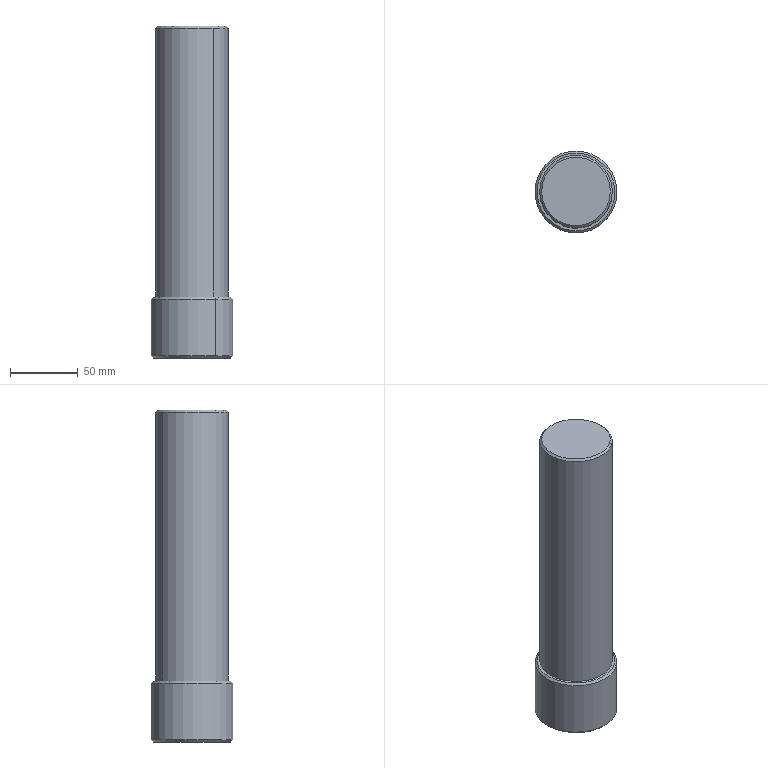Component | SolidWorks | PunchMandrel-1 | 1 solid | 13 faces | box 60.5 x 60.5 x 245 mm | volume 580883 mm3 | cone 6 | cylinder 4 | plane 3 | commonest cylinder face diameters 53.65 x2 60.5 x2
build123d program:
from build123d import *

# Parameters (mm, degrees)
CHAMFER1_SIZE = 1.5


with BuildPart() as part:
    # Sketch1 → Revolve1 (revolve)
    with BuildSketch(Plane.XY, mode=Mode.PRIVATE) as revolve1_sk:
        Polygon((0, 0), (0, 245), (30.25, 245), (30.25, 200), (26.825, 200), (26.825, 0), align=None)
    revolve(revolve1_sk.sketch.rotate(Axis((0, 0, 0), (0, 1, 0)), 90), axis=Axis((0, 0, 0), (0, 1, 0)))

    # Chamfer1
    chamfer1_edges = [part.edges().sort_by_distance(p)[0] for p in [
        (0, 0, 26.825),
        (0, 200, 30.25),
        (0, 245, 30.25),
    ]]
    chamfer(chamfer1_edges, length=CHAMFER1_SIZE)


solid = part.part

# Placed as in the assembly
solid = solid.moved(Location((0, 0, -1), (-90, 0, 0)))
STEP:
#1=COLOUR_RGB('',0.7922,0.8196,0.9333);
#2=FILL_AREA_STYLE_COLOUR('',#1);
#3=FILL_AREA_STYLE('',(#2));
#4=SURFACE_STYLE_FILL_AREA(#3);
#5=SURFACE_SIDE_STYLE('',(#4));
#6=SURFACE_STYLE_USAGE(.BOTH.,#5);
#7=PRESENTATION_STYLE_ASSIGNMENT((#6));
#8=CARTESIAN_POINT('',(0.6561,-0.9223,-7.913));
#9=VERTEX_POINT('',#8);
#10=CARTESIAN_POINT('',(-0.6561,0.9223,-7.913));
#11=VERTEX_POINT('',#10);
#12=CARTESIAN_POINT('',(-0.,-0.,-7.913));
#13=DIRECTION('',(0.,0.,1.));
#14=DIRECTION('',(0.5797,-0.8148,0.));
#15=AXIS2_PLACEMENT_3D('',#12,#13,#14);
#16=CIRCLE('',#15,1.132);
#17=EDGE_CURVE('',#9,#11,#16,.T.);
#18=ORIENTED_EDGE('',*,*,#17,.F.);
#19=CARTESIAN_POINT('',(0.6904,-0.9704,-7.972));
#20=VERTEX_POINT('',#19);
#21=CARTESIAN_POINT('',(0.6561,-0.9223,-7.913));
#22=DIRECTION('',(0.4099,-0.5762,-0.7071));
#23=VECTOR('',#22,39.37);
#24=LINE('',#21,#23);
#25=EDGE_CURVE('',#9,#20,#24,.T.);
#26=ORIENTED_EDGE('',*,*,#25,.T.);
#27=CARTESIAN_POINT('',(-0.6904,0.9704,-7.972));
#28=VERTEX_POINT('',#27);
#29=CARTESIAN_POINT('',(-0.,-0.,-7.972));
#30=DIRECTION('',(-0.,-0.,-1.));
#31=DIRECTION('',(0.5797,-0.8148,0.));
#32=AXIS2_PLACEMENT_3D('',#29,#30,#31);
#33=CIRCLE('',#32,1.191);
#34=EDGE_CURVE('',#28,#20,#33,.T.);
#35=ORIENTED_EDGE('',*,*,#34,.F.);
#36=CARTESIAN_POINT('',(-0.6561,0.9223,-7.913));
#37=DIRECTION('',(-0.4099,0.5762,-0.7071));
#38=VECTOR('',#37,39.37);
#39=LINE('',#36,#38);
#40=EDGE_CURVE('',#11,#28,#39,.T.);
#41=ORIENTED_EDGE('',*,*,#40,.F.);
#42=EDGE_LOOP('',(#18,#26,#35,#41));
#43=FACE_OUTER_BOUND('',#42,.T.);
#44=CARTESIAN_POINT('',(-0.,-0.,-7.913));
#45=DIRECTION('',(-0.,-0.,-1.));
#46=DIRECTION('',(-0.5797,0.8148,0.));
#47=AXIS2_PLACEMENT_3D('',#44,#45,#46);
#48=CONICAL_SURFACE('',#47,1.132,0.7854);
#49=ADVANCED_FACE('',(#43),#48,.T.);
#50=CARTESIAN_POINT('',(-0.6561,0.9223,-9.685));
#51=VERTEX_POINT('',#50);
#52=CARTESIAN_POINT('',(0.6561,-0.9223,-9.685));
#53=VERTEX_POINT('',#52);
#54=CARTESIAN_POINT('',(-0.,-0.,-9.685));
#55=DIRECTION('',(-0.,-0.,-1.));
#56=DIRECTION('',(-0.5797,0.8148,0.));
#57=AXIS2_PLACEMENT_3D('',#54,#55,#56);
#58=CIRCLE('',#57,1.132);
#59=EDGE_CURVE('',#51,#53,#58,.T.);
#60=ORIENTED_EDGE('',*,*,#59,.F.);
#61=CARTESIAN_POINT('',(-0.6904,0.9704,-9.626));
#62=VERTEX_POINT('',#61);
#63=CARTESIAN_POINT('',(-0.6904,0.9704,-9.626));
#64=DIRECTION('',(-0.4099,0.5762,0.7071));
#65=VECTOR('',#64,39.37);
#66=LINE('',#63,#65);
#67=EDGE_CURVE('',#51,#62,#66,.T.);
#68=ORIENTED_EDGE('',*,*,#67,.T.);
#69=CARTESIAN_POINT('',(0.6904,-0.9704,-9.626));
#70=VERTEX_POINT('',#69);
#71=CARTESIAN_POINT('',(-0.,-0.,-9.626));
#72=DIRECTION('',(0.,0.,1.));
#73=DIRECTION('',(-0.5797,0.8148,0.));
#74=AXIS2_PLACEMENT_3D('',#71,#72,#73);
#75=CIRCLE('',#74,1.191);
#76=EDGE_CURVE('',#70,#62,#75,.T.);
#77=ORIENTED_EDGE('',*,*,#76,.F.);
#78=CARTESIAN_POINT('',(0.6904,-0.9704,-9.626));
#79=DIRECTION('',(0.4099,-0.5762,0.7071));
#80=VECTOR('',#79,39.37);
#81=LINE('',#78,#80);
#82=EDGE_CURVE('',#53,#70,#81,.T.);
#83=ORIENTED_EDGE('',*,*,#82,.F.);
#84=EDGE_LOOP('',(#60,#68,#77,#83));
#85=FACE_OUTER_BOUND('',#84,.T.);
#86=CARTESIAN_POINT('',(-0.,-0.,-9.626));
#87=DIRECTION('',(0.,0.,1.));
#88=DIRECTION('',(0.5797,-0.8148,0.));
#89=AXIS2_PLACEMENT_3D('',#86,#87,#88);
#90=CONICAL_SURFACE('',#89,1.191,0.7854);
#91=ADVANCED_FACE('',(#85),#90,.T.);
#92=CARTESIAN_POINT('',(0.578,-0.8124,-0.03937));
#93=VERTEX_POINT('',#92);
#94=CARTESIAN_POINT('',(-0.578,0.8124,-0.03937));
#95=VERTEX_POINT('',#94);
#96=CARTESIAN_POINT('',(-0.,0.,-0.03937));
#97=DIRECTION('',(0.,0.,1.));
#98=DIRECTION('',(0.5797,-0.8148,0.));
#99=AXIS2_PLACEMENT_3D('',#96,#97,#98);
#100=CIRCLE('',#99,0.997);
#101=EDGE_CURVE('',#93,#95,#100,.T.);
#102=ORIENTED_EDGE('',*,*,#101,.F.);
#103=CARTESIAN_POINT('',(0.6122,-0.8606,-0.09843));
#104=VERTEX_POINT('',#103);
#105=CARTESIAN_POINT('',(0.578,-0.8124,-0.03937));
#106=DIRECTION('',(0.4099,-0.5762,-0.7071));
#107=VECTOR('',#106,39.37);
#108=LINE('',#105,#107);
#109=EDGE_CURVE('',#93,#104,#108,.T.);
#110=ORIENTED_EDGE('',*,*,#109,.T.);
#111=CARTESIAN_POINT('',(-0.6122,0.8606,-0.09843));
#112=VERTEX_POINT('',#111);
#113=CARTESIAN_POINT('',(-0.,0.,-0.09843));
#114=DIRECTION('',(-0.,-0.,-1.));
#115=DIRECTION('',(0.5797,-0.8148,0.));
#116=AXIS2_PLACEMENT_3D('',#113,#114,#115);
#117=CIRCLE('',#116,1.056);
#118=EDGE_CURVE('',#112,#104,#117,.T.);
#119=ORIENTED_EDGE('',*,*,#118,.F.);
#120=CARTESIAN_POINT('',(-0.578,0.8124,-0.03937));
#121=DIRECTION('',(-0.4099,0.5762,-0.7071));
#122=VECTOR('',#121,39.37);
#123=LINE('',#120,#122);
#124=EDGE_CURVE('',#95,#112,#123,.T.);
#125=ORIENTED_EDGE('',*,*,#124,.F.);
#126=EDGE_LOOP('',(#102,#110,#119,#125));
#127=FACE_OUTER_BOUND('',#126,.T.);
#128=CARTESIAN_POINT('',(-0.,0.,-0.03937));
#129=DIRECTION('',(-0.,-0.,-1.));
#130=DIRECTION('',(-0.5797,0.8148,-0.));
#131=AXIS2_PLACEMENT_3D('',#128,#129,#130);
#132=CONICAL_SURFACE('',#131,0.997,0.7854);
#133=ADVANCED_FACE('',(#127),#132,.T.);
#134=CARTESIAN_POINT('',(0.6122,-0.8606,-7.913));
#135=VERTEX_POINT('',#134);
#136=CARTESIAN_POINT('',(-0.6122,0.8606,-7.913));
#137=VERTEX_POINT('',#136);
#138=CARTESIAN_POINT('',(-0.,-0.,-7.913));
#139=DIRECTION('',(0.,0.,1.));
#140=DIRECTION('',(0.5797,-0.8148,0.));
#141=AXIS2_PLACEMENT_3D('',#138,#139,#140);
#142=CIRCLE('',#141,1.056);
#143=EDGE_CURVE('',#135,#137,#142,.T.);
#144=ORIENTED_EDGE('',*,*,#143,.T.);
#145=CARTESIAN_POINT('',(-0.6122,0.8606,-0.03937));
#146=DIRECTION('',(0.,0.,1.));
#147=VECTOR('',#146,39.37);
#148=LINE('',#145,#147);
#149=EDGE_CURVE('',#137,#112,#148,.T.);
#150=ORIENTED_EDGE('',*,*,#149,.T.);
#151=ORIENTED_EDGE('',*,*,#118,.T.);
#152=CARTESIAN_POINT('',(0.6122,-0.8606,-0.03937));
#153=DIRECTION('',(0.,0.,1.));
#154=VECTOR('',#153,39.37);
#155=LINE('',#152,#154);
#156=EDGE_CURVE('',#135,#104,#155,.T.);
#157=ORIENTED_EDGE('',*,*,#156,.F.);
#158=EDGE_LOOP('',(#144,#150,#151,#157));
#159=FACE_OUTER_BOUND('',#158,.T.);
#160=CARTESIAN_POINT('',(-0.,0.,-0.03937));
#161=DIRECTION('',(0.,0.,1.));
#162=DIRECTION('',(0.5797,-0.8148,0.));
#163=AXIS2_PLACEMENT_3D('',#160,#161,#162);
#164=CYLINDRICAL_SURFACE('',#163,1.056);
#165=ADVANCED_FACE('',(#159),#164,.T.);
#166=ORIENTED_EDGE('',*,*,#76,.T.);
#167=CARTESIAN_POINT('',(-0.6904,0.9704,-0.03937));
#168=DIRECTION('',(0.,0.,1.));
#169=VECTOR('',#168,39.37);
#170=LINE('',#167,#169);
#171=EDGE_CURVE('',#62,#28,#170,.T.);
#172=ORIENTED_EDGE('',*,*,#171,.T.);
#173=ORIENTED_EDGE('',*,*,#34,.T.);
#174=CARTESIAN_POINT('',(0.6904,-0.9704,-0.03937));
#175=DIRECTION('',(0.,0.,1.));
#176=VECTOR('',#175,39.37);
#177=LINE('',#174,#176);
#178=EDGE_CURVE('',#70,#20,#177,.T.);
#179=ORIENTED_EDGE('',*,*,#178,.F.);
#180=EDGE_LOOP('',(#166,#172,#173,#179));
#181=FACE_OUTER_BOUND('',#180,.T.);
#182=CARTESIAN_POINT('',(-0.,0.,-0.03937));
#183=DIRECTION('',(0.,0.,1.));
#184=DIRECTION('',(0.5797,-0.8148,0.));
#185=AXIS2_PLACEMENT_3D('',#182,#183,#184);
#186=CYLINDRICAL_SURFACE('',#185,1.191);
#187=ADVANCED_FACE('',(#181),#186,.T.);
#188=CARTESIAN_POINT('',(-0.,0.,-0.03937));
#189=DIRECTION('',(0.,0.,1.));
#190=DIRECTION('',(0.5797,-0.8148,0.));
#191=AXIS2_PLACEMENT_3D('',#188,#189,#190);
#192=CIRCLE('',#191,0.997);
#193=EDGE_CURVE('',#95,#93,#192,.T.);
#194=ORIENTED_EDGE('',*,*,#193,.T.);
#195=ORIENTED_EDGE('',*,*,#101,.T.);
#196=EDGE_LOOP('',(#194,#195));
#197=FACE_OUTER_BOUND('',#196,.T.);
#198=CARTESIAN_POINT('',(0.8606,0.6122,-0.03937));
#199=DIRECTION('',(0.,0.,1.));
#200=DIRECTION('',(0.5797,-0.8148,0.));
#201=AXIS2_PLACEMENT_3D('',#198,#199,#200);
#202=PLANE('',#201);
#203=ADVANCED_FACE('',(#197),#202,.T.);
#204=CARTESIAN_POINT('',(-0.,-0.,-9.685));
#205=DIRECTION('',(-0.,-0.,-1.));
#206=DIRECTION('',(-0.5797,0.8148,0.));
#207=AXIS2_PLACEMENT_3D('',#204,#205,#206);
#208=CIRCLE('',#207,1.132);
#209=EDGE_CURVE('',#53,#51,#208,.T.);
#210=ORIENTED_EDGE('',*,*,#209,.T.);
#211=ORIENTED_EDGE('',*,*,#59,.T.);
#212=EDGE_LOOP('',(#210,#211));
#213=FACE_OUTER_BOUND('',#212,.T.);
#214=CARTESIAN_POINT('',(-0.,-0.,-9.685));
#215=DIRECTION('',(-0.,-0.,-1.));
#216=DIRECTION('',(-0.5797,0.8148,-0.));
#217=AXIS2_PLACEMENT_3D('',#214,#215,#216);
#218=PLANE('',#217);
#219=ADVANCED_FACE('',(#213),#218,.T.);
#220=ORIENTED_EDGE('',*,*,#171,.F.);
#221=CARTESIAN_POINT('',(-0.,-0.,-9.626));
#222=DIRECTION('',(0.,0.,1.));
#223=DIRECTION('',(-0.5797,0.8148,0.));
#224=AXIS2_PLACEMENT_3D('',#221,#222,#223);
#225=CIRCLE('',#224,1.191);
#226=EDGE_CURVE('',#62,#70,#225,.T.);
#227=ORIENTED_EDGE('',*,*,#226,.T.);
#228=ORIENTED_EDGE('',*,*,#178,.T.);
#229=CARTESIAN_POINT('',(-0.,-0.,-7.972));
#230=DIRECTION('',(-0.,-0.,-1.));
#231=DIRECTION('',(0.5797,-0.8148,0.));
#232=AXIS2_PLACEMENT_3D('',#229,#230,#231);
#233=CIRCLE('',#232,1.191);
#234=EDGE_CURVE('',#20,#28,#233,.T.);
#235=ORIENTED_EDGE('',*,*,#234,.T.);
#236=EDGE_LOOP('',(#220,#227,#228,#235));
#237=FACE_OUTER_BOUND('',#236,.T.);
#238=CARTESIAN_POINT('',(-0.,0.,-0.03937));
#239=DIRECTION('',(0.,0.,1.));
#240=DIRECTION('',(0.5797,-0.8148,0.));
#241=AXIS2_PLACEMENT_3D('',#238,#239,#240);
#242=CYLINDRICAL_SURFACE('',#241,1.191);
#243=ADVANCED_FACE('',(#237),#242,.T.);
#244=CARTESIAN_POINT('',(-0.,-0.,-7.913));
#245=DIRECTION('',(0.,0.,1.));
#246=DIRECTION('',(0.5797,-0.8148,0.));
#247=AXIS2_PLACEMENT_3D('',#244,#245,#246);
#248=CIRCLE('',#247,1.132);
#249=EDGE_CURVE('',#11,#9,#248,.T.);
#250=ORIENTED_EDGE('',*,*,#249,.T.);
#251=ORIENTED_EDGE('',*,*,#17,.T.);
#252=EDGE_LOOP('',(#250,#251));
#253=FACE_OUTER_BOUND('',#252,.T.);
#254=ORIENTED_EDGE('',*,*,#143,.F.);
#255=CARTESIAN_POINT('',(-0.,-0.,-7.913));
#256=DIRECTION('',(0.,0.,1.));
#257=DIRECTION('',(0.5797,-0.8148,0.));
#258=AXIS2_PLACEMENT_3D('',#255,#256,#257);
#259=CIRCLE('',#258,1.056);
#260=EDGE_CURVE('',#137,#135,#259,.T.);
#261=ORIENTED_EDGE('',*,*,#260,.F.);
#262=EDGE_LOOP('',(#254,#261));
#263=FACE_BOUND('',#262,.T.);
#264=CARTESIAN_POINT('',(0.9704,0.6904,-7.913));
#265=DIRECTION('',(0.,0.,1.));
#266=DIRECTION('',(0.5797,-0.8148,0.));
#267=AXIS2_PLACEMENT_3D('',#264,#265,#266);
#268=PLANE('',#267);
#269=ADVANCED_FACE('',(#253,#263),#268,.T.);
#270=ORIENTED_EDGE('',*,*,#149,.F.);
#271=ORIENTED_EDGE('',*,*,#260,.T.);
#272=ORIENTED_EDGE('',*,*,#156,.T.);
#273=CARTESIAN_POINT('',(-0.,0.,-0.09843));
#274=DIRECTION('',(-0.,-0.,-1.));
#275=DIRECTION('',(0.5797,-0.8148,0.));
#276=AXIS2_PLACEMENT_3D('',#273,#274,#275);
#277=CIRCLE('',#276,1.056);
#278=EDGE_CURVE('',#104,#112,#277,.T.);
#279=ORIENTED_EDGE('',*,*,#278,.T.);
#280=EDGE_LOOP('',(#270,#271,#272,#279));
#281=FACE_OUTER_BOUND('',#280,.T.);
#282=CARTESIAN_POINT('',(-0.,0.,-0.03937));
#283=DIRECTION('',(0.,0.,1.));
#284=DIRECTION('',(0.5797,-0.8148,0.));
#285=AXIS2_PLACEMENT_3D('',#282,#283,#284);
#286=CYLINDRICAL_SURFACE('',#285,1.056);
#287=ADVANCED_FACE('',(#281),#286,.T.);
#288=ORIENTED_EDGE('',*,*,#109,.F.);
#289=ORIENTED_EDGE('',*,*,#193,.F.);
#290=ORIENTED_EDGE('',*,*,#124,.T.);
#291=ORIENTED_EDGE('',*,*,#278,.F.);
#292=EDGE_LOOP('',(#288,#289,#290,#291));
#293=FACE_OUTER_BOUND('',#292,.T.);
#294=CARTESIAN_POINT('',(-0.,0.,-0.03937));
#295=DIRECTION('',(-0.,-0.,-1.));
#296=DIRECTION('',(-0.5797,0.8148,-0.));
#297=AXIS2_PLACEMENT_3D('',#294,#295,#296);
#298=CONICAL_SURFACE('',#297,0.997,0.7854);
#299=ADVANCED_FACE('',(#293),#298,.T.);
#300=ORIENTED_EDGE('',*,*,#67,.F.);
#301=ORIENTED_EDGE('',*,*,#209,.F.);
#302=ORIENTED_EDGE('',*,*,#82,.T.);
#303=ORIENTED_EDGE('',*,*,#226,.F.);
#304=EDGE_LOOP('',(#300,#301,#302,#303));
#305=FACE_OUTER_BOUND('',#304,.T.);
#306=CARTESIAN_POINT('',(-0.,-0.,-9.626));
#307=DIRECTION('',(0.,0.,1.));
#308=DIRECTION('',(0.5797,-0.8148,0.));
#309=AXIS2_PLACEMENT_3D('',#306,#307,#308);
#310=CONICAL_SURFACE('',#309,1.191,0.7854);
#311=ADVANCED_FACE('',(#305),#310,.T.);
#312=ORIENTED_EDGE('',*,*,#25,.F.);
#313=ORIENTED_EDGE('',*,*,#249,.F.);
#314=ORIENTED_EDGE('',*,*,#40,.T.);
#315=ORIENTED_EDGE('',*,*,#234,.F.);
#316=EDGE_LOOP('',(#312,#313,#314,#315));
#317=FACE_OUTER_BOUND('',#316,.T.);
#318=CARTESIAN_POINT('',(-0.,-0.,-7.913));
#319=DIRECTION('',(-0.,-0.,-1.));
#320=DIRECTION('',(-0.5797,0.8148,0.));
#321=AXIS2_PLACEMENT_3D('',#318,#319,#320);
#322=CONICAL_SURFACE('',#321,1.132,0.7854);
#323=ADVANCED_FACE('',(#317),#322,.T.);
#324=CLOSED_SHELL('',(#49,#91,#133,#165,#187,#203,#219,#243,#269,#287,#299,#311,#323));
#325=MANIFOLD_SOLID_BREP('',#324);
#326=STYLED_ITEM('',(#7),#325);
#327=(LENGTH_UNIT()NAMED_UNIT(*)SI_UNIT($,.METRE.));
#328=LENGTH_MEASURE_WITH_UNIT(LENGTH_MEASURE(0.0254),#327);
#329=DIMENSIONAL_EXPONENTS(1.,0.,0.,0.,0.,0.,0.);
#330=(CONVERSION_BASED_UNIT('',#328)LENGTH_UNIT()NAMED_UNIT(#329));
#331=UNCERTAINTY_MEASURE_WITH_UNIT(LENGTH_MEASURE(0.00001),#330,'','');
#332=(NAMED_UNIT(*)PLANE_ANGLE_UNIT()SI_UNIT($,.RADIAN.));
#333=(NAMED_UNIT(*)SI_UNIT($,.STERADIAN.)SOLID_ANGLE_UNIT());
#334=(GEOMETRIC_REPRESENTATION_CONTEXT(3)GLOBAL_UNCERTAINTY_ASSIGNED_CONTEXT((#331))GLOBAL_UNIT_ASSIGNED_CONTEXT((#330,#332,#333))REPRESENTATION_CONTEXT('',''));
#335=MECHANICAL_DESIGN_GEOMETRIC_PRESENTATION_REPRESENTATION('',(#326),#334);
#336=PRESENTATION_LAYER_ASSIGNMENT('','',(#326));
#337=CARTESIAN_POINT('',(0.,0.,0.));
#338=DIRECTION('',(0.,0.,1.));
#339=DIRECTION('',(1.,0.,0.));
#340=AXIS2_PLACEMENT_3D('',#337,#338,#339);
#341=(LENGTH_UNIT()NAMED_UNIT(*)SI_UNIT($,.METRE.));
#342=LENGTH_MEASURE_WITH_UNIT(LENGTH_MEASURE(0.0254),#341);
#343=DIMENSIONAL_EXPONENTS(1.,0.,0.,0.,0.,0.,0.);
#344=(CONVERSION_BASED_UNIT('',#342)LENGTH_UNIT()NAMED_UNIT(#343));
#345=UNCERTAINTY_MEASURE_WITH_UNIT(LENGTH_MEASURE(0.00001),#344,'','');
#346=(NAMED_UNIT(*)PLANE_ANGLE_UNIT()SI_UNIT($,.RADIAN.));
#347=(NAMED_UNIT(*)SI_UNIT($,.STERADIAN.)SOLID_ANGLE_UNIT());
#348=(GEOMETRIC_REPRESENTATION_CONTEXT(3)GLOBAL_UNCERTAINTY_ASSIGNED_CONTEXT((#345))GLOBAL_UNIT_ASSIGNED_CONTEXT((#344,#346,#347))REPRESENTATION_CONTEXT('',''));
#349=ADVANCED_BREP_SHAPE_REPRESENTATION('',(#325,#340),#348);